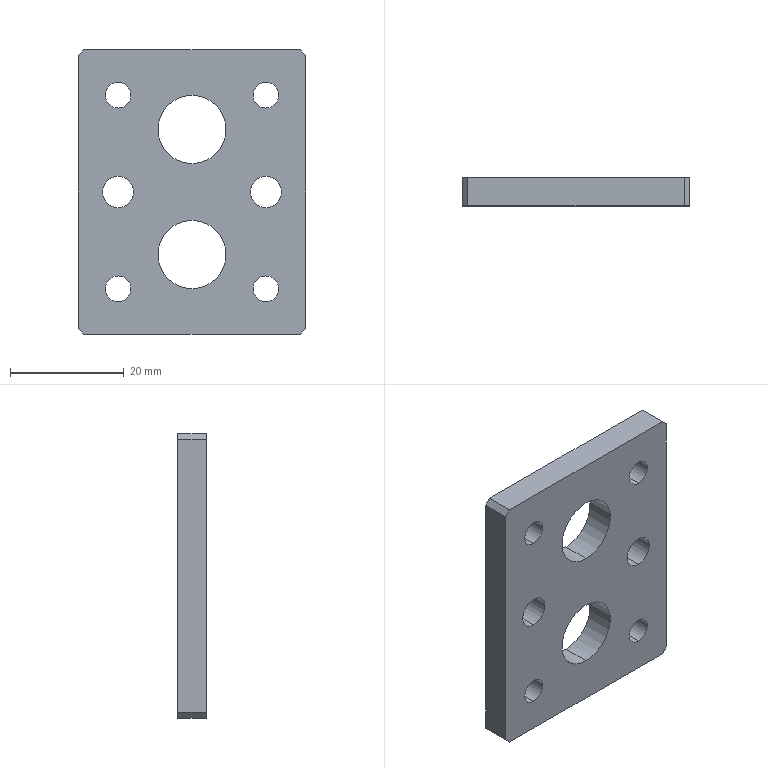Component | SolidWorks | DZ.KX.203-TC1505-30-09-01-05-08-1 | 1 solid | 26 faces | box 40 x 5 x 50 mm | volume 8303 mm3 | cylinder 16 | plane 10 | commonest cylinder face diameters 4.5 x8 5.5 x4 12 x4
build123d program:
from build123d import *

# Parameters (mm, degrees)
SKETCH1_W                  = 50
SKETCH1_H                  = 40
BOSS_EXTRUDE1_DEPTH        = 5
F_4_5_4_5_DIAMETER_HOLE1_D = 4.5
F_12_0_12_DIAMETER_HOLE1_D = 12
CHAMFER2_SIZE              = 1
F_5_5_5_5_DIAMETER_HOLE1_D = 5.5


with BuildPart() as part:
    # Sketch1 → Boss-Extrude1 (new body)
    with BuildSketch(Plane(origin=(0, 0, 0), x_dir=(0, 0, -1), z_dir=(1, 0, 0))):
        Rectangle(SKETCH1_W, SKETCH1_H)
    extrude(amount=BOSS_EXTRUDE1_DEPTH)

    # 4.5 _4.5_ Diameter Hole1 (through all)
    with Locations(Plane.ZY):
        with Locations((-17, 13), (17, 13), (17, -13), (-17, -13)):
            Hole(F_4_5_4_5_DIAMETER_HOLE1_D / 2)

    # 12.0 _12_ Diameter Hole1 (through all)
    with Locations(Plane.ZY):
        with Locations((-11, 0), (11, 0)):
            Hole(F_12_0_12_DIAMETER_HOLE1_D / 2)

    # Chamfer2
    chamfer2_edges = [part.edges().sort_by_distance(p)[0] for p in [
        (2.5, 20, 25),
        (2.5, 20, -25),
        (2.5, -20, -25),
        (2.5, -20, 25),
    ]]
    chamfer(chamfer2_edges, length=CHAMFER2_SIZE)

    # 5.5 _5.5_ Diameter Hole1 (through all)
    with Locations(Plane.ZY):
        with Locations((0, 13), (0, -13)):
            Hole(F_5_5_5_5_DIAMETER_HOLE1_D / 2)


solid = part.part

# Placed as in the assembly
solid = solid.moved(Location((294.5, -650.807, -11.94), (0, 0, 90)))
STEP:
#1=COLOUR_RGB('',0.7922,0.8196,0.9333);
#2=FILL_AREA_STYLE_COLOUR('',#1);
#3=FILL_AREA_STYLE('',(#2));
#4=SURFACE_STYLE_FILL_AREA(#3);
#5=SURFACE_SIDE_STYLE('',(#4));
#6=SURFACE_STYLE_USAGE(.BOTH.,#5);
#7=PRESENTATION_STYLE_ASSIGNMENT((#6));
#8=CARTESIAN_POINT('',(11.083,-25.425,-0.5784));
#9=VERTEX_POINT('',#8);
#10=CARTESIAN_POINT('',(11.083,-25.425,-0.3618));
#11=VERTEX_POINT('',#10);
#12=CARTESIAN_POINT('',(11.083,-25.425,-0.4701));
#13=DIRECTION('',(0.,-1.,-0.));
#14=DIRECTION('',(0.,0.,1.));
#15=AXIS2_PLACEMENT_3D('',#12,#13,#14);
#16=CIRCLE('',#15,0.1083);
#17=EDGE_CURVE('',#9,#11,#16,.T.);
#18=ORIENTED_EDGE('',*,*,#17,.F.);
#19=CARTESIAN_POINT('',(11.083,-25.622,-0.5784));
#20=VERTEX_POINT('',#19);
#21=CARTESIAN_POINT('',(11.083,-25.622,-0.5784));
#22=DIRECTION('',(0.,-1.,-0.));
#23=VECTOR('',#22,39.37);
#24=LINE('',#21,#23);
#25=EDGE_CURVE('',#9,#20,#24,.T.);
#26=ORIENTED_EDGE('',*,*,#25,.T.);
#27=CARTESIAN_POINT('',(11.083,-25.622,-0.3618));
#28=VERTEX_POINT('',#27);
#29=CARTESIAN_POINT('',(11.083,-25.622,-0.4701));
#30=DIRECTION('',(0.,-1.,-0.));
#31=DIRECTION('',(0.,0.,1.));
#32=AXIS2_PLACEMENT_3D('',#29,#30,#31);
#33=CIRCLE('',#32,0.1083);
#34=EDGE_CURVE('',#20,#28,#33,.T.);
#35=ORIENTED_EDGE('',*,*,#34,.T.);
#36=CARTESIAN_POINT('',(11.083,-25.622,-0.3618));
#37=DIRECTION('',(0.,-1.,-0.));
#38=VECTOR('',#37,39.37);
#39=LINE('',#36,#38);
#40=EDGE_CURVE('',#11,#28,#39,.T.);
#41=ORIENTED_EDGE('',*,*,#40,.F.);
#42=EDGE_LOOP('',(#18,#26,#35,#41));
#43=FACE_OUTER_BOUND('',#42,.T.);
#44=CARTESIAN_POINT('',(11.083,-25.622,-0.4701));
#45=DIRECTION('',(0.,-1.,-0.));
#46=DIRECTION('',(0.,0.,1.));
#47=AXIS2_PLACEMENT_3D('',#44,#45,#46);
#48=CYLINDRICAL_SURFACE('',#47,0.1083);
#49=ADVANCED_FACE('',(#43),#48,.F.);
#50=CARTESIAN_POINT('',(12.106,-25.425,-0.5784));
#51=VERTEX_POINT('',#50);
#52=CARTESIAN_POINT('',(12.106,-25.425,-0.3618));
#53=VERTEX_POINT('',#52);
#54=CARTESIAN_POINT('',(12.106,-25.425,-0.4701));
#55=DIRECTION('',(0.,-1.,-0.));
#56=DIRECTION('',(0.,0.,1.));
#57=AXIS2_PLACEMENT_3D('',#54,#55,#56);
#58=CIRCLE('',#57,0.1083);
#59=EDGE_CURVE('',#51,#53,#58,.T.);
#60=ORIENTED_EDGE('',*,*,#59,.F.);
#61=CARTESIAN_POINT('',(12.106,-25.622,-0.5784));
#62=VERTEX_POINT('',#61);
#63=CARTESIAN_POINT('',(12.106,-25.622,-0.5784));
#64=DIRECTION('',(0.,-1.,-0.));
#65=VECTOR('',#64,39.37);
#66=LINE('',#63,#65);
#67=EDGE_CURVE('',#51,#62,#66,.T.);
#68=ORIENTED_EDGE('',*,*,#67,.T.);
#69=CARTESIAN_POINT('',(12.106,-25.622,-0.3618));
#70=VERTEX_POINT('',#69);
#71=CARTESIAN_POINT('',(12.106,-25.622,-0.4701));
#72=DIRECTION('',(0.,-1.,-0.));
#73=DIRECTION('',(0.,0.,1.));
#74=AXIS2_PLACEMENT_3D('',#71,#72,#73);
#75=CIRCLE('',#74,0.1083);
#76=EDGE_CURVE('',#62,#70,#75,.T.);
#77=ORIENTED_EDGE('',*,*,#76,.T.);
#78=CARTESIAN_POINT('',(12.106,-25.622,-0.3618));
#79=DIRECTION('',(0.,-1.,-0.));
#80=VECTOR('',#79,39.37);
#81=LINE('',#78,#80);
#82=EDGE_CURVE('',#53,#70,#81,.T.);
#83=ORIENTED_EDGE('',*,*,#82,.F.);
#84=EDGE_LOOP('',(#60,#68,#77,#83));
#85=FACE_OUTER_BOUND('',#84,.T.);
#86=CARTESIAN_POINT('',(12.106,-25.622,-0.4701));
#87=DIRECTION('',(0.,-1.,-0.));
#88=DIRECTION('',(0.,0.,1.));
#89=AXIS2_PLACEMENT_3D('',#86,#87,#88);
#90=CYLINDRICAL_SURFACE('',#89,0.1083);
#91=ADVANCED_FACE('',(#85),#90,.F.);
#92=CARTESIAN_POINT('',(11.594,-25.425,-1.139));
#93=VERTEX_POINT('',#92);
#94=CARTESIAN_POINT('',(11.594,-25.425,-0.6669));
#95=VERTEX_POINT('',#94);
#96=CARTESIAN_POINT('',(11.594,-25.425,-0.9032));
#97=DIRECTION('',(0.,-1.,-0.));
#98=DIRECTION('',(0.,0.,1.));
#99=AXIS2_PLACEMENT_3D('',#96,#97,#98);
#100=CIRCLE('',#99,0.2362);
#101=EDGE_CURVE('',#93,#95,#100,.T.);
#102=ORIENTED_EDGE('',*,*,#101,.F.);
#103=CARTESIAN_POINT('',(11.594,-25.622,-1.139));
#104=VERTEX_POINT('',#103);
#105=CARTESIAN_POINT('',(11.594,-25.622,-1.139));
#106=DIRECTION('',(0.,-1.,-0.));
#107=VECTOR('',#106,39.37);
#108=LINE('',#105,#107);
#109=EDGE_CURVE('',#93,#104,#108,.T.);
#110=ORIENTED_EDGE('',*,*,#109,.T.);
#111=CARTESIAN_POINT('',(11.594,-25.622,-0.6669));
#112=VERTEX_POINT('',#111);
#113=CARTESIAN_POINT('',(11.594,-25.622,-0.9032));
#114=DIRECTION('',(0.,-1.,-0.));
#115=DIRECTION('',(0.,0.,1.));
#116=AXIS2_PLACEMENT_3D('',#113,#114,#115);
#117=CIRCLE('',#116,0.2362);
#118=EDGE_CURVE('',#104,#112,#117,.T.);
#119=ORIENTED_EDGE('',*,*,#118,.T.);
#120=CARTESIAN_POINT('',(11.594,-25.622,-0.6669));
#121=DIRECTION('',(0.,-1.,-0.));
#122=VECTOR('',#121,39.37);
#123=LINE('',#120,#122);
#124=EDGE_CURVE('',#95,#112,#123,.T.);
#125=ORIENTED_EDGE('',*,*,#124,.F.);
#126=EDGE_LOOP('',(#102,#110,#119,#125));
#127=FACE_OUTER_BOUND('',#126,.T.);
#128=CARTESIAN_POINT('',(11.594,-25.622,-0.9032));
#129=DIRECTION('',(0.,-1.,-0.));
#130=DIRECTION('',(0.,0.,1.));
#131=AXIS2_PLACEMENT_3D('',#128,#129,#130);
#132=CYLINDRICAL_SURFACE('',#131,0.2362);
#133=ADVANCED_FACE('',(#127),#132,.F.);
#134=CARTESIAN_POINT('',(11.594,-25.425,-0.2732));
#135=VERTEX_POINT('',#134);
#136=CARTESIAN_POINT('',(11.594,-25.425,0.1992));
#137=VERTEX_POINT('',#136);
#138=CARTESIAN_POINT('',(11.594,-25.425,-0.03703));
#139=DIRECTION('',(0.,-1.,-0.));
#140=DIRECTION('',(0.,0.,1.));
#141=AXIS2_PLACEMENT_3D('',#138,#139,#140);
#142=CIRCLE('',#141,0.2362);
#143=EDGE_CURVE('',#135,#137,#142,.T.);
#144=ORIENTED_EDGE('',*,*,#143,.F.);
#145=CARTESIAN_POINT('',(11.594,-25.622,-0.2732));
#146=VERTEX_POINT('',#145);
#147=CARTESIAN_POINT('',(11.594,-25.622,-0.2732));
#148=DIRECTION('',(0.,-1.,-0.));
#149=VECTOR('',#148,39.37);
#150=LINE('',#147,#149);
#151=EDGE_CURVE('',#135,#146,#150,.T.);
#152=ORIENTED_EDGE('',*,*,#151,.T.);
#153=CARTESIAN_POINT('',(11.594,-25.622,0.1992));
#154=VERTEX_POINT('',#153);
#155=CARTESIAN_POINT('',(11.594,-25.622,-0.03703));
#156=DIRECTION('',(0.,-1.,-0.));
#157=DIRECTION('',(0.,0.,1.));
#158=AXIS2_PLACEMENT_3D('',#155,#156,#157);
#159=CIRCLE('',#158,0.2362);
#160=EDGE_CURVE('',#146,#154,#159,.T.);
#161=ORIENTED_EDGE('',*,*,#160,.T.);
#162=CARTESIAN_POINT('',(11.594,-25.622,0.1992));
#163=DIRECTION('',(0.,-1.,-0.));
#164=VECTOR('',#163,39.37);
#165=LINE('',#162,#164);
#166=EDGE_CURVE('',#137,#154,#165,.T.);
#167=ORIENTED_EDGE('',*,*,#166,.F.);
#168=EDGE_LOOP('',(#144,#152,#161,#167));
#169=FACE_OUTER_BOUND('',#168,.T.);
#170=CARTESIAN_POINT('',(11.594,-25.622,-0.03703));
#171=DIRECTION('',(0.,-1.,-0.));
#172=DIRECTION('',(0.,0.,1.));
#173=AXIS2_PLACEMENT_3D('',#170,#171,#172);
#174=CYLINDRICAL_SURFACE('',#173,0.2362);
#175=ADVANCED_FACE('',(#169),#174,.F.);
#176=CARTESIAN_POINT('',(11.083,-25.425,-1.228));
#177=VERTEX_POINT('',#176);
#178=CARTESIAN_POINT('',(11.083,-25.425,-1.051));
#179=VERTEX_POINT('',#178);
#180=CARTESIAN_POINT('',(11.083,-25.425,-1.139));
#181=DIRECTION('',(0.,-1.,-0.));
#182=DIRECTION('',(0.,0.,1.));
#183=AXIS2_PLACEMENT_3D('',#180,#181,#182);
#184=CIRCLE('',#183,0.08858);
#185=EDGE_CURVE('',#177,#179,#184,.T.);
#186=ORIENTED_EDGE('',*,*,#185,.F.);
#187=CARTESIAN_POINT('',(11.083,-25.622,-1.228));
#188=VERTEX_POINT('',#187);
#189=CARTESIAN_POINT('',(11.083,-25.622,-1.228));
#190=DIRECTION('',(0.,-1.,-0.));
#191=VECTOR('',#190,39.37);
#192=LINE('',#189,#191);
#193=EDGE_CURVE('',#177,#188,#192,.T.);
#194=ORIENTED_EDGE('',*,*,#193,.T.);
#195=CARTESIAN_POINT('',(11.083,-25.622,-1.051));
#196=VERTEX_POINT('',#195);
#197=CARTESIAN_POINT('',(11.083,-25.622,-1.139));
#198=DIRECTION('',(0.,-1.,-0.));
#199=DIRECTION('',(0.,0.,1.));
#200=AXIS2_PLACEMENT_3D('',#197,#198,#199);
#201=CIRCLE('',#200,0.08858);
#202=EDGE_CURVE('',#188,#196,#201,.T.);
#203=ORIENTED_EDGE('',*,*,#202,.T.);
#204=CARTESIAN_POINT('',(11.083,-25.622,-1.051));
#205=DIRECTION('',(0.,-1.,-0.));
#206=VECTOR('',#205,39.37);
#207=LINE('',#204,#206);
#208=EDGE_CURVE('',#179,#196,#207,.T.);
#209=ORIENTED_EDGE('',*,*,#208,.F.);
#210=EDGE_LOOP('',(#186,#194,#203,#209));
#211=FACE_OUTER_BOUND('',#210,.T.);
#212=CARTESIAN_POINT('',(11.083,-25.622,-1.139));
#213=DIRECTION('',(0.,-1.,-0.));
#214=DIRECTION('',(0.,0.,1.));
#215=AXIS2_PLACEMENT_3D('',#212,#213,#214);
#216=CYLINDRICAL_SURFACE('',#215,0.08858);
#217=ADVANCED_FACE('',(#211),#216,.F.);
#218=CARTESIAN_POINT('',(11.083,-25.425,0.1106));
#219=VERTEX_POINT('',#218);
#220=CARTESIAN_POINT('',(11.083,-25.425,0.2878));
#221=VERTEX_POINT('',#220);
#222=CARTESIAN_POINT('',(11.083,-25.425,0.1992));
#223=DIRECTION('',(0.,-1.,-0.));
#224=DIRECTION('',(0.,0.,1.));
#225=AXIS2_PLACEMENT_3D('',#222,#223,#224);
#226=CIRCLE('',#225,0.08858);
#227=EDGE_CURVE('',#219,#221,#226,.T.);
#228=ORIENTED_EDGE('',*,*,#227,.F.);
#229=CARTESIAN_POINT('',(11.083,-25.622,0.1106));
#230=VERTEX_POINT('',#229);
#231=CARTESIAN_POINT('',(11.083,-25.622,0.1106));
#232=DIRECTION('',(0.,-1.,-0.));
#233=VECTOR('',#232,39.37);
#234=LINE('',#231,#233);
#235=EDGE_CURVE('',#219,#230,#234,.T.);
#236=ORIENTED_EDGE('',*,*,#235,.T.);
#237=CARTESIAN_POINT('',(11.083,-25.622,0.2878));
#238=VERTEX_POINT('',#237);
#239=CARTESIAN_POINT('',(11.083,-25.622,0.1992));
#240=DIRECTION('',(0.,-1.,-0.));
#241=DIRECTION('',(0.,0.,1.));
#242=AXIS2_PLACEMENT_3D('',#239,#240,#241);
#243=CIRCLE('',#242,0.08858);
#244=EDGE_CURVE('',#230,#238,#243,.T.);
#245=ORIENTED_EDGE('',*,*,#244,.T.);
#246=CARTESIAN_POINT('',(11.083,-25.622,0.2878));
#247=DIRECTION('',(0.,-1.,-0.));
#248=VECTOR('',#247,39.37);
#249=LINE('',#246,#248);
#250=EDGE_CURVE('',#221,#238,#249,.T.);
#251=ORIENTED_EDGE('',*,*,#250,.F.);
#252=EDGE_LOOP('',(#228,#236,#245,#251));
#253=FACE_OUTER_BOUND('',#252,.T.);
#254=CARTESIAN_POINT('',(11.083,-25.622,0.1992));
#255=DIRECTION('',(0.,-1.,-0.));
#256=DIRECTION('',(0.,0.,1.));
#257=AXIS2_PLACEMENT_3D('',#254,#255,#256);
#258=CYLINDRICAL_SURFACE('',#257,0.08858);
#259=ADVANCED_FACE('',(#253),#258,.F.);
#260=CARTESIAN_POINT('',(12.106,-25.425,0.1106));
#261=VERTEX_POINT('',#260);
#262=CARTESIAN_POINT('',(12.106,-25.425,0.2878));
#263=VERTEX_POINT('',#262);
#264=CARTESIAN_POINT('',(12.106,-25.425,0.1992));
#265=DIRECTION('',(0.,-1.,-0.));
#266=DIRECTION('',(0.,0.,1.));
#267=AXIS2_PLACEMENT_3D('',#264,#265,#266);
#268=CIRCLE('',#267,0.08858);
#269=EDGE_CURVE('',#261,#263,#268,.T.);
#270=ORIENTED_EDGE('',*,*,#269,.F.);
#271=CARTESIAN_POINT('',(12.106,-25.622,0.1106));
#272=VERTEX_POINT('',#271);
#273=CARTESIAN_POINT('',(12.106,-25.622,0.1106));
#274=DIRECTION('',(0.,-1.,-0.));
#275=VECTOR('',#274,39.37);
#276=LINE('',#273,#275);
#277=EDGE_CURVE('',#261,#272,#276,.T.);
#278=ORIENTED_EDGE('',*,*,#277,.T.);
#279=CARTESIAN_POINT('',(12.106,-25.622,0.2878));
#280=VERTEX_POINT('',#279);
#281=CARTESIAN_POINT('',(12.106,-25.622,0.1992));
#282=DIRECTION('',(0.,-1.,-0.));
#283=DIRECTION('',(0.,0.,1.));
#284=AXIS2_PLACEMENT_3D('',#281,#282,#283);
#285=CIRCLE('',#284,0.08858);
#286=EDGE_CURVE('',#272,#280,#285,.T.);
#287=ORIENTED_EDGE('',*,*,#286,.T.);
#288=CARTESIAN_POINT('',(12.106,-25.622,0.2878));
#289=DIRECTION('',(0.,-1.,-0.));
#290=VECTOR('',#289,39.37);
#291=LINE('',#288,#290);
#292=EDGE_CURVE('',#263,#280,#291,.T.);
#293=ORIENTED_EDGE('',*,*,#292,.F.);
#294=EDGE_LOOP('',(#270,#278,#287,#293));
#295=FACE_OUTER_BOUND('',#294,.T.);
#296=CARTESIAN_POINT('',(12.106,-25.622,0.1992));
#297=DIRECTION('',(0.,-1.,-0.));
#298=DIRECTION('',(0.,0.,1.));
#299=AXIS2_PLACEMENT_3D('',#296,#297,#298);
#300=CYLINDRICAL_SURFACE('',#299,0.08858);
#301=ADVANCED_FACE('',(#295),#300,.F.);
#302=CARTESIAN_POINT('',(12.106,-25.425,-1.228));
#303=VERTEX_POINT('',#302);
#304=CARTESIAN_POINT('',(12.106,-25.425,-1.051));
#305=VERTEX_POINT('',#304);
#306=CARTESIAN_POINT('',(12.106,-25.425,-1.139));
#307=DIRECTION('',(0.,-1.,-0.));
#308=DIRECTION('',(0.,0.,1.));
#309=AXIS2_PLACEMENT_3D('',#306,#307,#308);
#310=CIRCLE('',#309,0.08858);
#311=EDGE_CURVE('',#303,#305,#310,.T.);
#312=ORIENTED_EDGE('',*,*,#311,.F.);
#313=CARTESIAN_POINT('',(12.106,-25.622,-1.228));
#314=VERTEX_POINT('',#313);
#315=CARTESIAN_POINT('',(12.106,-25.622,-1.228));
#316=DIRECTION('',(0.,-1.,-0.));
#317=VECTOR('',#316,39.37);
#318=LINE('',#315,#317);
#319=EDGE_CURVE('',#303,#314,#318,.T.);
#320=ORIENTED_EDGE('',*,*,#319,.T.);
#321=CARTESIAN_POINT('',(12.106,-25.622,-1.051));
#322=VERTEX_POINT('',#321);
#323=CARTESIAN_POINT('',(12.106,-25.622,-1.139));
#324=DIRECTION('',(0.,-1.,-0.));
#325=DIRECTION('',(0.,0.,1.));
#326=AXIS2_PLACEMENT_3D('',#323,#324,#325);
#327=CIRCLE('',#326,0.08858);
#328=EDGE_CURVE('',#314,#322,#327,.T.);
#329=ORIENTED_EDGE('',*,*,#328,.T.);
#330=CARTESIAN_POINT('',(12.106,-25.622,-1.051));
#331=DIRECTION('',(0.,-1.,-0.));
#332=VECTOR('',#331,39.37);
#333=LINE('',#330,#332);
#334=EDGE_CURVE('',#305,#322,#333,.T.);
#335=ORIENTED_EDGE('',*,*,#334,.F.);
#336=EDGE_LOOP('',(#312,#320,#329,#335));
#337=FACE_OUTER_BOUND('',#336,.T.);
#338=CARTESIAN_POINT('',(12.106,-25.622,-1.139));
#339=DIRECTION('',(0.,-1.,-0.));
#340=DIRECTION('',(0.,0.,1.));
#341=AXIS2_PLACEMENT_3D('',#338,#339,#340);
#342=CYLINDRICAL_SURFACE('',#341,0.08858);
#343=ADVANCED_FACE('',(#337),#342,.F.);
#344=CARTESIAN_POINT('',(10.846,-25.425,0.5142));
#345=VERTEX_POINT('',#344);
#346=CARTESIAN_POINT('',(12.343,-25.425,0.5142));
#347=VERTEX_POINT('',#346);
#348=CARTESIAN_POINT('',(12.382,-25.425,0.5142));
#349=DIRECTION('',(1.,0.,0.));
#350=VECTOR('',#349,39.37);
#351=LINE('',#348,#350);
#352=EDGE_CURVE('',#345,#347,#351,.T.);
#353=ORIENTED_EDGE('',*,*,#352,.F.);
#354=CARTESIAN_POINT('',(10.846,-25.622,0.5142));
#355=VERTEX_POINT('',#354);
#356=CARTESIAN_POINT('',(10.846,-25.425,0.5142));
#357=DIRECTION('',(0.,-1.,-0.));
#358=VECTOR('',#357,39.37);
#359=LINE('',#356,#358);
#360=EDGE_CURVE('',#345,#355,#359,.T.);
#361=ORIENTED_EDGE('',*,*,#360,.T.);
#362=CARTESIAN_POINT('',(12.343,-25.622,0.5142));
#363=VERTEX_POINT('',#362);
#364=CARTESIAN_POINT('',(12.382,-25.622,0.5142));
#365=DIRECTION('',(1.,0.,0.));
#366=VECTOR('',#365,39.37);
#367=LINE('',#364,#366);
#368=EDGE_CURVE('',#355,#363,#367,.T.);
#369=ORIENTED_EDGE('',*,*,#368,.T.);
#370=CARTESIAN_POINT('',(12.343,-25.425,0.5142));
#371=DIRECTION('',(-0.,1.,0.));
#372=VECTOR('',#371,39.37);
#373=LINE('',#370,#372);
#374=EDGE_CURVE('',#363,#347,#373,.T.);
#375=ORIENTED_EDGE('',*,*,#374,.T.);
#376=EDGE_LOOP('',(#353,#361,#369,#375));
#377=FACE_OUTER_BOUND('',#376,.T.);
#378=CARTESIAN_POINT('',(12.382,-25.425,0.5142));
#379=DIRECTION('',(0.,0.,-1.));
#380=DIRECTION('',(0.,-1.,-0.));
#381=AXIS2_PLACEMENT_3D('',#378,#379,#380);
#382=PLANE('',#381);
#383=ADVANCED_FACE('',(#377),#382,.F.);
#384=CARTESIAN_POINT('',(12.382,-25.425,0.4748));
#385=VERTEX_POINT('',#384);
#386=CARTESIAN_POINT('',(12.382,-25.425,-1.415));
#387=VERTEX_POINT('',#386);
#388=CARTESIAN_POINT('',(12.382,-25.425,-1.454));
#389=DIRECTION('',(-0.,0.,-1.));
#390=VECTOR('',#389,39.37);
#391=LINE('',#388,#390);
#392=EDGE_CURVE('',#385,#387,#391,.T.);
#393=ORIENTED_EDGE('',*,*,#392,.F.);
#394=CARTESIAN_POINT('',(12.382,-25.622,0.4748));
#395=VERTEX_POINT('',#394);
#396=CARTESIAN_POINT('',(12.382,-25.425,0.4748));
#397=DIRECTION('',(0.,-1.,-0.));
#398=VECTOR('',#397,39.37);
#399=LINE('',#396,#398);
#400=EDGE_CURVE('',#385,#395,#399,.T.);
#401=ORIENTED_EDGE('',*,*,#400,.T.);
#402=CARTESIAN_POINT('',(12.382,-25.622,-1.415));
#403=VERTEX_POINT('',#402);
#404=CARTESIAN_POINT('',(12.382,-25.622,-1.454));
#405=DIRECTION('',(-0.,0.,-1.));
#406=VECTOR('',#405,39.37);
#407=LINE('',#404,#406);
#408=EDGE_CURVE('',#395,#403,#407,.T.);
#409=ORIENTED_EDGE('',*,*,#408,.T.);
#410=CARTESIAN_POINT('',(12.382,-25.425,-1.415));
#411=DIRECTION('',(-0.,1.,0.));
#412=VECTOR('',#411,39.37);
#413=LINE('',#410,#412);
#414=EDGE_CURVE('',#403,#387,#413,.T.);
#415=ORIENTED_EDGE('',*,*,#414,.T.);
#416=EDGE_LOOP('',(#393,#401,#409,#415));
#417=FACE_OUTER_BOUND('',#416,.T.);
#418=CARTESIAN_POINT('',(12.382,-25.425,-1.454));
#419=DIRECTION('',(-1.,-0.,0.));
#420=DIRECTION('',(0.,-0.,1.));
#421=AXIS2_PLACEMENT_3D('',#418,#419,#420);
#422=PLANE('',#421);
#423=ADVANCED_FACE('',(#417),#422,.F.);
#424=CARTESIAN_POINT('',(12.343,-25.622,-1.454));
#425=VERTEX_POINT('',#424);
#426=CARTESIAN_POINT('',(10.846,-25.622,-1.454));
#427=VERTEX_POINT('',#426);
#428=CARTESIAN_POINT('',(12.382,-25.622,-1.454));
#429=DIRECTION('',(-1.,-0.,-0.));
#430=VECTOR('',#429,39.37);
#431=LINE('',#428,#430);
#432=EDGE_CURVE('',#425,#427,#431,.T.);
#433=ORIENTED_EDGE('',*,*,#432,.T.);
#434=CARTESIAN_POINT('',(10.846,-25.425,-1.454));
#435=VERTEX_POINT('',#434);
#436=CARTESIAN_POINT('',(10.846,-25.425,-1.454));
#437=DIRECTION('',(-0.,1.,0.));
#438=VECTOR('',#437,39.37);
#439=LINE('',#436,#438);
#440=EDGE_CURVE('',#427,#435,#439,.T.);
#441=ORIENTED_EDGE('',*,*,#440,.T.);
#442=CARTESIAN_POINT('',(12.343,-25.425,-1.454));
#443=VERTEX_POINT('',#442);
#444=CARTESIAN_POINT('',(12.382,-25.425,-1.454));
#445=DIRECTION('',(-1.,-0.,-0.));
#446=VECTOR('',#445,39.37);
#447=LINE('',#444,#446);
#448=EDGE_CURVE('',#443,#435,#447,.T.);
#449=ORIENTED_EDGE('',*,*,#448,.F.);
#450=CARTESIAN_POINT('',(12.343,-25.425,-1.454));
#451=DIRECTION('',(0.,-1.,-0.));
#452=VECTOR('',#451,39.37);
#453=LINE('',#450,#452);
#454=EDGE_CURVE('',#443,#425,#453,.T.);
#455=ORIENTED_EDGE('',*,*,#454,.T.);
#456=EDGE_LOOP('',(#433,#441,#449,#455));
#457=FACE_OUTER_BOUND('',#456,.T.);
#458=CARTESIAN_POINT('',(12.382,-25.425,-1.454));
#459=DIRECTION('',(-0.,-0.,1.));
#460=DIRECTION('',(-0.,1.,0.));
#461=AXIS2_PLACEMENT_3D('',#458,#459,#460);
#462=PLANE('',#461);
#463=ADVANCED_FACE('',(#457),#462,.F.);
#464=CARTESIAN_POINT('',(10.807,-25.622,-1.415));
#465=VERTEX_POINT('',#464);
#466=CARTESIAN_POINT('',(10.807,-25.622,0.4748));
#467=VERTEX_POINT('',#466);
#468=CARTESIAN_POINT('',(10.807,-25.622,-1.454));
#469=DIRECTION('',(0.,-0.,1.));
#470=VECTOR('',#469,39.37);
#471=LINE('',#468,#470);
#472=EDGE_CURVE('',#465,#467,#471,.T.);
#473=ORIENTED_EDGE('',*,*,#472,.T.);
#474=CARTESIAN_POINT('',(10.807,-25.425,0.4748));
#475=VERTEX_POINT('',#474);
#476=CARTESIAN_POINT('',(10.807,-25.425,0.4748));
#477=DIRECTION('',(-0.,1.,0.));
#478=VECTOR('',#477,39.37);
#479=LINE('',#476,#478);
#480=EDGE_CURVE('',#467,#475,#479,.T.);
#481=ORIENTED_EDGE('',*,*,#480,.T.);
#482=CARTESIAN_POINT('',(10.807,-25.425,-1.415));
#483=VERTEX_POINT('',#482);
#484=CARTESIAN_POINT('',(10.807,-25.425,-1.454));
#485=DIRECTION('',(0.,-0.,1.));
#486=VECTOR('',#485,39.37);
#487=LINE('',#484,#486);
#488=EDGE_CURVE('',#483,#475,#487,.T.);
#489=ORIENTED_EDGE('',*,*,#488,.F.);
#490=CARTESIAN_POINT('',(10.807,-25.425,-1.415));
#491=DIRECTION('',(0.,-1.,-0.));
#492=VECTOR('',#491,39.37);
#493=LINE('',#490,#492);
#494=EDGE_CURVE('',#483,#465,#493,.T.);
#495=ORIENTED_EDGE('',*,*,#494,.T.);
#496=EDGE_LOOP('',(#473,#481,#489,#495));
#497=FACE_OUTER_BOUND('',#496,.T.);
#498=CARTESIAN_POINT('',(10.807,-25.425,-1.454));
#499=DIRECTION('',(1.,0.,-0.));
#500=DIRECTION('',(-0.,0.,-1.));
#501=AXIS2_PLACEMENT_3D('',#498,#499,#500);
#502=PLANE('',#501);
#503=ADVANCED_FACE('',(#497),#502,.F.);
#504=CARTESIAN_POINT('',(11.083,-25.425,-0.4701));
#505=DIRECTION('',(0.,-1.,-0.));
#506=DIRECTION('',(0.,0.,1.));
#507=AXIS2_PLACEMENT_3D('',#504,#505,#506);
#508=CIRCLE('',#507,0.1083);
#509=EDGE_CURVE('',#11,#9,#508,.T.);
#510=ORIENTED_EDGE('',*,*,#509,.T.);
#511=ORIENTED_EDGE('',*,*,#17,.T.);
#512=EDGE_LOOP('',(#510,#511));
#513=FACE_BOUND('',#512,.T.);
#514=CARTESIAN_POINT('',(12.106,-25.425,-0.4701));
#515=DIRECTION('',(0.,-1.,-0.));
#516=DIRECTION('',(0.,0.,1.));
#517=AXIS2_PLACEMENT_3D('',#514,#515,#516);
#518=CIRCLE('',#517,0.1083);
#519=EDGE_CURVE('',#53,#51,#518,.T.);
#520=ORIENTED_EDGE('',*,*,#519,.T.);
#521=ORIENTED_EDGE('',*,*,#59,.T.);
#522=EDGE_LOOP('',(#520,#521));
#523=FACE_BOUND('',#522,.T.);
#524=CARTESIAN_POINT('',(11.594,-25.425,-0.9032));
#525=DIRECTION('',(0.,-1.,-0.));
#526=DIRECTION('',(0.,0.,1.));
#527=AXIS2_PLACEMENT_3D('',#524,#525,#526);
#528=CIRCLE('',#527,0.2362);
#529=EDGE_CURVE('',#95,#93,#528,.T.);
#530=ORIENTED_EDGE('',*,*,#529,.T.);
#531=ORIENTED_EDGE('',*,*,#101,.T.);
#532=EDGE_LOOP('',(#530,#531));
#533=FACE_BOUND('',#532,.T.);
#534=CARTESIAN_POINT('',(11.594,-25.425,-0.03703));
#535=DIRECTION('',(0.,-1.,-0.));
#536=DIRECTION('',(0.,0.,1.));
#537=AXIS2_PLACEMENT_3D('',#534,#535,#536);
#538=CIRCLE('',#537,0.2362);
#539=EDGE_CURVE('',#137,#135,#538,.T.);
#540=ORIENTED_EDGE('',*,*,#539,.T.);
#541=ORIENTED_EDGE('',*,*,#143,.T.);
#542=EDGE_LOOP('',(#540,#541));
#543=FACE_BOUND('',#542,.T.);
#544=CARTESIAN_POINT('',(11.083,-25.425,-1.139));
#545=DIRECTION('',(0.,-1.,-0.));
#546=DIRECTION('',(0.,0.,1.));
#547=AXIS2_PLACEMENT_3D('',#544,#545,#546);
#548=CIRCLE('',#547,0.08858);
#549=EDGE_CURVE('',#179,#177,#548,.T.);
#550=ORIENTED_EDGE('',*,*,#549,.T.);
#551=ORIENTED_EDGE('',*,*,#185,.T.);
#552=EDGE_LOOP('',(#550,#551));
#553=FACE_BOUND('',#552,.T.);
#554=CARTESIAN_POINT('',(11.083,-25.425,0.1992));
#555=DIRECTION('',(0.,-1.,-0.));
#556=DIRECTION('',(0.,0.,1.));
#557=AXIS2_PLACEMENT_3D('',#554,#555,#556);
#558=CIRCLE('',#557,0.08858);
#559=EDGE_CURVE('',#221,#219,#558,.T.);
#560=ORIENTED_EDGE('',*,*,#559,.T.);
#561=ORIENTED_EDGE('',*,*,#227,.T.);
#562=EDGE_LOOP('',(#560,#561));
#563=FACE_BOUND('',#562,.T.);
#564=CARTESIAN_POINT('',(12.106,-25.425,0.1992));
#565=DIRECTION('',(0.,-1.,-0.));
#566=DIRECTION('',(0.,0.,1.));
#567=AXIS2_PLACEMENT_3D('',#564,#565,#566);
#568=CIRCLE('',#567,0.08858);
#569=EDGE_CURVE('',#263,#261,#568,.T.);
#570=ORIENTED_EDGE('',*,*,#569,.T.);
#571=ORIENTED_EDGE('',*,*,#269,.T.);
#572=EDGE_LOOP('',(#570,#571));
#573=FACE_BOUND('',#572,.T.);
#574=CARTESIAN_POINT('',(12.106,-25.425,-1.139));
#575=DIRECTION('',(0.,-1.,-0.));
#576=DIRECTION('',(0.,0.,1.));
#577=AXIS2_PLACEMENT_3D('',#574,#575,#576);
#578=CIRCLE('',#577,0.08858);
#579=EDGE_CURVE('',#305,#303,#578,.T.);
#580=ORIENTED_EDGE('',*,*,#579,.T.);
#581=ORIENTED_EDGE('',*,*,#311,.T.);
#582=EDGE_LOOP('',(#580,#581));
#583=FACE_BOUND('',#582,.T.);
#584=ORIENTED_EDGE('',*,*,#488,.T.);
#585=CARTESIAN_POINT('',(10.728,-25.425,0.396));
#586=DIRECTION('',(0.7071,0.,0.7071));
#587=VECTOR('',#586,39.37);
#588=LINE('',#585,#587);
#589=EDGE_CURVE('',#475,#345,#588,.T.);
#590=ORIENTED_EDGE('',*,*,#589,.T.);
#591=ORIENTED_EDGE('',*,*,#352,.T.);
#592=CARTESIAN_POINT('',(12.461,-25.425,0.396));
#593=DIRECTION('',(0.7071,0.,-0.7071));
#594=VECTOR('',#593,39.37);
#595=LINE('',#592,#594);
#596=EDGE_CURVE('',#347,#385,#595,.T.);
#597=ORIENTED_EDGE('',*,*,#596,.T.);
#598=ORIENTED_EDGE('',*,*,#392,.T.);
#599=CARTESIAN_POINT('',(12.461,-25.425,-1.336));
#600=DIRECTION('',(-0.7071,-0.,-0.7071));
#601=VECTOR('',#600,39.37);
#602=LINE('',#599,#601);
#603=EDGE_CURVE('',#387,#443,#602,.T.);
#604=ORIENTED_EDGE('',*,*,#603,.T.);
#605=ORIENTED_EDGE('',*,*,#448,.T.);
#606=CARTESIAN_POINT('',(10.728,-25.425,-1.336));
#607=DIRECTION('',(-0.7071,-0.,0.7071));
#608=VECTOR('',#607,39.37);
#609=LINE('',#606,#608);
#610=EDGE_CURVE('',#435,#483,#609,.T.);
#611=ORIENTED_EDGE('',*,*,#610,.T.);
#612=EDGE_LOOP('',(#584,#590,#591,#597,#598,#604,#605,#611));
#613=FACE_OUTER_BOUND('',#612,.T.);
#614=CARTESIAN_POINT('',(11.594,-25.425,-0.4701));
#615=DIRECTION('',(-0.,1.,0.));
#616=DIRECTION('',(0.,0.,-1.));
#617=AXIS2_PLACEMENT_3D('',#614,#615,#616);
#618=PLANE('',#617);
#619=ADVANCED_FACE('',(#513,#523,#533,#543,#553,#563,#573,#583,#613),#618,.T.);
#620=CARTESIAN_POINT('',(11.083,-25.622,-0.4701));
#621=DIRECTION('',(0.,-1.,-0.));
#622=DIRECTION('',(0.,0.,1.));
#623=AXIS2_PLACEMENT_3D('',#620,#621,#622);
#624=CIRCLE('',#623,0.1083);
#625=EDGE_CURVE('',#28,#20,#624,.T.);
#626=ORIENTED_EDGE('',*,*,#625,.F.);
#627=ORIENTED_EDGE('',*,*,#34,.F.);
#628=EDGE_LOOP('',(#626,#627));
#629=FACE_BOUND('',#628,.T.);
#630=CARTESIAN_POINT('',(12.106,-25.622,-0.4701));
#631=DIRECTION('',(0.,-1.,-0.));
#632=DIRECTION('',(0.,0.,1.));
#633=AXIS2_PLACEMENT_3D('',#630,#631,#632);
#634=CIRCLE('',#633,0.1083);
#635=EDGE_CURVE('',#70,#62,#634,.T.);
#636=ORIENTED_EDGE('',*,*,#635,.F.);
#637=ORIENTED_EDGE('',*,*,#76,.F.);
#638=EDGE_LOOP('',(#636,#637));
#639=FACE_BOUND('',#638,.T.);
#640=CARTESIAN_POINT('',(11.594,-25.622,-0.9032));
#641=DIRECTION('',(0.,-1.,-0.));
#642=DIRECTION('',(0.,0.,1.));
#643=AXIS2_PLACEMENT_3D('',#640,#641,#642);
#644=CIRCLE('',#643,0.2362);
#645=EDGE_CURVE('',#112,#104,#644,.T.);
#646=ORIENTED_EDGE('',*,*,#645,.F.);
#647=ORIENTED_EDGE('',*,*,#118,.F.);
#648=EDGE_LOOP('',(#646,#647));
#649=FACE_BOUND('',#648,.T.);
#650=CARTESIAN_POINT('',(11.594,-25.622,-0.03703));
#651=DIRECTION('',(0.,-1.,-0.));
#652=DIRECTION('',(0.,0.,1.));
#653=AXIS2_PLACEMENT_3D('',#650,#651,#652);
#654=CIRCLE('',#653,0.2362);
#655=EDGE_CURVE('',#154,#146,#654,.T.);
#656=ORIENTED_EDGE('',*,*,#655,.F.);
#657=ORIENTED_EDGE('',*,*,#160,.F.);
#658=EDGE_LOOP('',(#656,#657));
#659=FACE_BOUND('',#658,.T.);
#660=CARTESIAN_POINT('',(11.083,-25.622,-1.139));
#661=DIRECTION('',(0.,-1.,-0.));
#662=DIRECTION('',(0.,0.,1.));
#663=AXIS2_PLACEMENT_3D('',#660,#661,#662);
#664=CIRCLE('',#663,0.08858);
#665=EDGE_CURVE('',#196,#188,#664,.T.);
#666=ORIENTED_EDGE('',*,*,#665,.F.);
#667=ORIENTED_EDGE('',*,*,#202,.F.);
#668=EDGE_LOOP('',(#666,#667));
#669=FACE_BOUND('',#668,.T.);
#670=CARTESIAN_POINT('',(11.083,-25.622,0.1992));
#671=DIRECTION('',(0.,-1.,-0.));
#672=DIRECTION('',(0.,0.,1.));
#673=AXIS2_PLACEMENT_3D('',#670,#671,#672);
#674=CIRCLE('',#673,0.08858);
#675=EDGE_CURVE('',#238,#230,#674,.T.);
#676=ORIENTED_EDGE('',*,*,#675,.F.);
#677=ORIENTED_EDGE('',*,*,#244,.F.);
#678=EDGE_LOOP('',(#676,#677));
#679=FACE_BOUND('',#678,.T.);
#680=CARTESIAN_POINT('',(12.106,-25.622,0.1992));
#681=DIRECTION('',(0.,-1.,-0.));
#682=DIRECTION('',(0.,0.,1.));
#683=AXIS2_PLACEMENT_3D('',#680,#681,#682);
#684=CIRCLE('',#683,0.08858);
#685=EDGE_CURVE('',#280,#272,#684,.T.);
#686=ORIENTED_EDGE('',*,*,#685,.F.);
#687=ORIENTED_EDGE('',*,*,#286,.F.);
#688=EDGE_LOOP('',(#686,#687));
#689=FACE_BOUND('',#688,.T.);
#690=CARTESIAN_POINT('',(12.106,-25.622,-1.139));
#691=DIRECTION('',(0.,-1.,-0.));
#692=DIRECTION('',(0.,0.,1.));
#693=AXIS2_PLACEMENT_3D('',#690,#691,#692);
#694=CIRCLE('',#693,0.08858);
#695=EDGE_CURVE('',#322,#314,#694,.T.);
#696=ORIENTED_EDGE('',*,*,#695,.F.);
#697=ORIENTED_EDGE('',*,*,#328,.F.);
#698=EDGE_LOOP('',(#696,#697));
#699=FACE_BOUND('',#698,.T.);
#700=ORIENTED_EDGE('',*,*,#368,.F.);
#701=CARTESIAN_POINT('',(10.846,-25.622,0.5142));
#702=DIRECTION('',(-0.7071,-0.,-0.7071));
#703=VECTOR('',#702,39.37);
#704=LINE('',#701,#703);
#705=EDGE_CURVE('',#355,#467,#704,.T.);
#706=ORIENTED_EDGE('',*,*,#705,.T.);
#707=ORIENTED_EDGE('',*,*,#472,.F.);
#708=CARTESIAN_POINT('',(10.807,-25.622,-1.415));
#709=DIRECTION('',(0.7071,0.,-0.7071));
#710=VECTOR('',#709,39.37);
#711=LINE('',#708,#710);
#712=EDGE_CURVE('',#465,#427,#711,.T.);
#713=ORIENTED_EDGE('',*,*,#712,.T.);
#714=ORIENTED_EDGE('',*,*,#432,.F.);
#715=CARTESIAN_POINT('',(12.343,-25.622,-1.454));
#716=DIRECTION('',(0.7071,0.,0.7071));
#717=VECTOR('',#716,39.37);
#718=LINE('',#715,#717);
#719=EDGE_CURVE('',#425,#403,#718,.T.);
#720=ORIENTED_EDGE('',*,*,#719,.T.);
#721=ORIENTED_EDGE('',*,*,#408,.F.);
#722=CARTESIAN_POINT('',(12.382,-25.622,0.4748));
#723=DIRECTION('',(-0.7071,-0.,0.7071));
#724=VECTOR('',#723,39.37);
#725=LINE('',#722,#724);
#726=EDGE_CURVE('',#395,#363,#725,.T.);
#727=ORIENTED_EDGE('',*,*,#726,.T.);
#728=EDGE_LOOP('',(#700,#706,#707,#713,#714,#720,#721,#727));
#729=FACE_OUTER_BOUND('',#728,.T.);
#730=CARTESIAN_POINT('',(11.594,-25.622,-0.4701));
#731=DIRECTION('',(-0.,1.,0.));
#732=DIRECTION('',(0.,0.,-1.));
#733=AXIS2_PLACEMENT_3D('',#730,#731,#732);
#734=PLANE('',#733);
#735=ADVANCED_FACE('',(#629,#639,#649,#659,#669,#679,#689,#699,#729),#734,.F.);
#736=ORIENTED_EDGE('',*,*,#319,.F.);
#737=ORIENTED_EDGE('',*,*,#579,.F.);
#738=ORIENTED_EDGE('',*,*,#334,.T.);
#739=ORIENTED_EDGE('',*,*,#695,.T.);
#740=EDGE_LOOP('',(#736,#737,#738,#739));
#741=FACE_OUTER_BOUND('',#740,.T.);
#742=CARTESIAN_POINT('',(12.106,-25.622,-1.139));
#743=DIRECTION('',(0.,-1.,-0.));
#744=DIRECTION('',(0.,0.,1.));
#745=AXIS2_PLACEMENT_3D('',#742,#743,#744);
#746=CYLINDRICAL_SURFACE('',#745,0.08858);
#747=ADVANCED_FACE('',(#741),#746,.F.);
#748=ORIENTED_EDGE('',*,*,#277,.F.);
#749=ORIENTED_EDGE('',*,*,#569,.F.);
#750=ORIENTED_EDGE('',*,*,#292,.T.);
#751=ORIENTED_EDGE('',*,*,#685,.T.);
#752=EDGE_LOOP('',(#748,#749,#750,#751));
#753=FACE_OUTER_BOUND('',#752,.T.);
#754=CARTESIAN_POINT('',(12.106,-25.622,0.1992));
#755=DIRECTION('',(0.,-1.,-0.));
#756=DIRECTION('',(0.,0.,1.));
#757=AXIS2_PLACEMENT_3D('',#754,#755,#756);
#758=CYLINDRICAL_SURFACE('',#757,0.08858);
#759=ADVANCED_FACE('',(#753),#758,.F.);
#760=ORIENTED_EDGE('',*,*,#235,.F.);
#761=ORIENTED_EDGE('',*,*,#559,.F.);
#762=ORIENTED_EDGE('',*,*,#250,.T.);
#763=ORIENTED_EDGE('',*,*,#675,.T.);
#764=EDGE_LOOP('',(#760,#761,#762,#763));
#765=FACE_OUTER_BOUND('',#764,.T.);
#766=CARTESIAN_POINT('',(11.083,-25.622,0.1992));
#767=DIRECTION('',(0.,-1.,-0.));
#768=DIRECTION('',(0.,0.,1.));
#769=AXIS2_PLACEMENT_3D('',#766,#767,#768);
#770=CYLINDRICAL_SURFACE('',#769,0.08858);
#771=ADVANCED_FACE('',(#765),#770,.F.);
#772=ORIENTED_EDGE('',*,*,#193,.F.);
#773=ORIENTED_EDGE('',*,*,#549,.F.);
#774=ORIENTED_EDGE('',*,*,#208,.T.);
#775=ORIENTED_EDGE('',*,*,#665,.T.);
#776=EDGE_LOOP('',(#772,#773,#774,#775));
#777=FACE_OUTER_BOUND('',#776,.T.);
#778=CARTESIAN_POINT('',(11.083,-25.622,-1.139));
#779=DIRECTION('',(0.,-1.,-0.));
#780=DIRECTION('',(0.,0.,1.));
#781=AXIS2_PLACEMENT_3D('',#778,#779,#780);
#782=CYLINDRICAL_SURFACE('',#781,0.08858);
#783=ADVANCED_FACE('',(#777),#782,.F.);
#784=ORIENTED_EDGE('',*,*,#151,.F.);
#785=ORIENTED_EDGE('',*,*,#539,.F.);
#786=ORIENTED_EDGE('',*,*,#166,.T.);
#787=ORIENTED_EDGE('',*,*,#655,.T.);
#788=EDGE_LOOP('',(#784,#785,#786,#787));
#789=FACE_OUTER_BOUND('',#788,.T.);
#790=CARTESIAN_POINT('',(11.594,-25.622,-0.03703));
#791=DIRECTION('',(0.,-1.,-0.));
#792=DIRECTION('',(0.,0.,1.));
#793=AXIS2_PLACEMENT_3D('',#790,#791,#792);
#794=CYLINDRICAL_SURFACE('',#793,0.2362);
#795=ADVANCED_FACE('',(#789),#794,.F.);
#796=ORIENTED_EDGE('',*,*,#109,.F.);
#797=ORIENTED_EDGE('',*,*,#529,.F.);
#798=ORIENTED_EDGE('',*,*,#124,.T.);
#799=ORIENTED_EDGE('',*,*,#645,.T.);
#800=EDGE_LOOP('',(#796,#797,#798,#799));
#801=FACE_OUTER_BOUND('',#800,.T.);
#802=CARTESIAN_POINT('',(11.594,-25.622,-0.9032));
#803=DIRECTION('',(0.,-1.,-0.));
#804=DIRECTION('',(0.,0.,1.));
#805=AXIS2_PLACEMENT_3D('',#802,#803,#804);
#806=CYLINDRICAL_SURFACE('',#805,0.2362);
#807=ADVANCED_FACE('',(#801),#806,.F.);
#808=ORIENTED_EDGE('',*,*,#589,.F.);
#809=ORIENTED_EDGE('',*,*,#480,.F.);
#810=ORIENTED_EDGE('',*,*,#705,.F.);
#811=ORIENTED_EDGE('',*,*,#360,.F.);
#812=EDGE_LOOP('',(#808,#809,#810,#811));
#813=FACE_OUTER_BOUND('',#812,.T.);
#814=CARTESIAN_POINT('',(10.846,-25.425,0.5142));
#815=DIRECTION('',(0.7071,0.,-0.7071));
#816=DIRECTION('',(0.,-1.,-0.));
#817=AXIS2_PLACEMENT_3D('',#814,#815,#816);
#818=PLANE('',#817);
#819=ADVANCED_FACE('',(#813),#818,.F.);
#820=ORIENTED_EDGE('',*,*,#596,.F.);
#821=ORIENTED_EDGE('',*,*,#374,.F.);
#822=ORIENTED_EDGE('',*,*,#726,.F.);
#823=ORIENTED_EDGE('',*,*,#400,.F.);
#824=EDGE_LOOP('',(#820,#821,#822,#823));
#825=FACE_OUTER_BOUND('',#824,.T.);
#826=CARTESIAN_POINT('',(12.382,-25.425,0.4748));
#827=DIRECTION('',(-0.7071,-0.,-0.7071));
#828=DIRECTION('',(0.,-1.,-0.));
#829=AXIS2_PLACEMENT_3D('',#826,#827,#828);
#830=PLANE('',#829);
#831=ADVANCED_FACE('',(#825),#830,.F.);
#832=ORIENTED_EDGE('',*,*,#610,.F.);
#833=ORIENTED_EDGE('',*,*,#440,.F.);
#834=ORIENTED_EDGE('',*,*,#712,.F.);
#835=ORIENTED_EDGE('',*,*,#494,.F.);
#836=EDGE_LOOP('',(#832,#833,#834,#835));
#837=FACE_OUTER_BOUND('',#836,.T.);
#838=CARTESIAN_POINT('',(10.807,-25.425,-1.415));
#839=DIRECTION('',(0.7071,0.,0.7071));
#840=DIRECTION('',(0.,-1.,-0.));
#841=AXIS2_PLACEMENT_3D('',#838,#839,#840);
#842=PLANE('',#841);
#843=ADVANCED_FACE('',(#837),#842,.F.);
#844=ORIENTED_EDGE('',*,*,#603,.F.);
#845=ORIENTED_EDGE('',*,*,#414,.F.);
#846=ORIENTED_EDGE('',*,*,#719,.F.);
#847=ORIENTED_EDGE('',*,*,#454,.F.);
#848=EDGE_LOOP('',(#844,#845,#846,#847));
#849=FACE_OUTER_BOUND('',#848,.T.);
#850=CARTESIAN_POINT('',(12.343,-25.425,-1.454));
#851=DIRECTION('',(-0.7071,-0.,0.7071));
#852=DIRECTION('',(0.,-1.,-0.));
#853=AXIS2_PLACEMENT_3D('',#850,#851,#852);
#854=PLANE('',#853);
#855=ADVANCED_FACE('',(#849),#854,.F.);
#856=ORIENTED_EDGE('',*,*,#67,.F.);
#857=ORIENTED_EDGE('',*,*,#519,.F.);
#858=ORIENTED_EDGE('',*,*,#82,.T.);
#859=ORIENTED_EDGE('',*,*,#635,.T.);
#860=EDGE_LOOP('',(#856,#857,#858,#859));
#861=FACE_OUTER_BOUND('',#860,.T.);
#862=CARTESIAN_POINT('',(12.106,-25.622,-0.4701));
#863=DIRECTION('',(0.,-1.,-0.));
#864=DIRECTION('',(0.,0.,1.));
#865=AXIS2_PLACEMENT_3D('',#862,#863,#864);
#866=CYLINDRICAL_SURFACE('',#865,0.1083);
#867=ADVANCED_FACE('',(#861),#866,.F.);
#868=ORIENTED_EDGE('',*,*,#25,.F.);
#869=ORIENTED_EDGE('',*,*,#509,.F.);
#870=ORIENTED_EDGE('',*,*,#40,.T.);
#871=ORIENTED_EDGE('',*,*,#625,.T.);
#872=EDGE_LOOP('',(#868,#869,#870,#871));
#873=FACE_OUTER_BOUND('',#872,.T.);
#874=CARTESIAN_POINT('',(11.083,-25.622,-0.4701));
#875=DIRECTION('',(0.,-1.,-0.));
#876=DIRECTION('',(0.,0.,1.));
#877=AXIS2_PLACEMENT_3D('',#874,#875,#876);
#878=CYLINDRICAL_SURFACE('',#877,0.1083);
#879=ADVANCED_FACE('',(#873),#878,.F.);
#880=CLOSED_SHELL('',(#49,#91,#133,#175,#217,#259,#301,#343,#383,#423,#463,#503,#619,#735,#747,#759,#771,#783,#795,#807,#819,#831,#843,#855,#867,#879));
#881=MANIFOLD_SOLID_BREP('',#880);
#882=STYLED_ITEM('',(#7),#881);
#883=(LENGTH_UNIT()NAMED_UNIT(*)SI_UNIT($,.METRE.));
#884=LENGTH_MEASURE_WITH_UNIT(LENGTH_MEASURE(0.0254),#883);
#885=DIMENSIONAL_EXPONENTS(1.,0.,0.,0.,0.,0.,0.);
#886=(CONVERSION_BASED_UNIT('',#884)LENGTH_UNIT()NAMED_UNIT(#885));
#887=UNCERTAINTY_MEASURE_WITH_UNIT(LENGTH_MEASURE(0.00001),#886,'','');
#888=(NAMED_UNIT(*)PLANE_ANGLE_UNIT()SI_UNIT($,.RADIAN.));
#889=(NAMED_UNIT(*)SI_UNIT($,.STERADIAN.)SOLID_ANGLE_UNIT());
#890=(GEOMETRIC_REPRESENTATION_CONTEXT(3)GLOBAL_UNCERTAINTY_ASSIGNED_CONTEXT((#887))GLOBAL_UNIT_ASSIGNED_CONTEXT((#886,#888,#889))REPRESENTATION_CONTEXT('',''));
#891=MECHANICAL_DESIGN_GEOMETRIC_PRESENTATION_REPRESENTATION('',(#882),#890);
#892=CARTESIAN_POINT('',(0.,0.,0.));
#893=DIRECTION('',(0.,0.,1.));
#894=DIRECTION('',(1.,0.,0.));
#895=AXIS2_PLACEMENT_3D('',#892,#893,#894);
#896=(LENGTH_UNIT()NAMED_UNIT(*)SI_UNIT($,.METRE.));
#897=LENGTH_MEASURE_WITH_UNIT(LENGTH_MEASURE(0.0254),#896);
#898=DIMENSIONAL_EXPONENTS(1.,0.,0.,0.,0.,0.,0.);
#899=(CONVERSION_BASED_UNIT('',#897)LENGTH_UNIT()NAMED_UNIT(#898));
#900=UNCERTAINTY_MEASURE_WITH_UNIT(LENGTH_MEASURE(0.00001),#899,'','');
#901=(NAMED_UNIT(*)PLANE_ANGLE_UNIT()SI_UNIT($,.RADIAN.));
#902=(NAMED_UNIT(*)SI_UNIT($,.STERADIAN.)SOLID_ANGLE_UNIT());
#903=(GEOMETRIC_REPRESENTATION_CONTEXT(3)GLOBAL_UNCERTAINTY_ASSIGNED_CONTEXT((#900))GLOBAL_UNIT_ASSIGNED_CONTEXT((#899,#901,#902))REPRESENTATION_CONTEXT('',''));
#904=ADVANCED_BREP_SHAPE_REPRESENTATION('',(#881,#895),#903);
#905=PRESENTATION_LAYER_ASSIGNMENT('','',(#882));